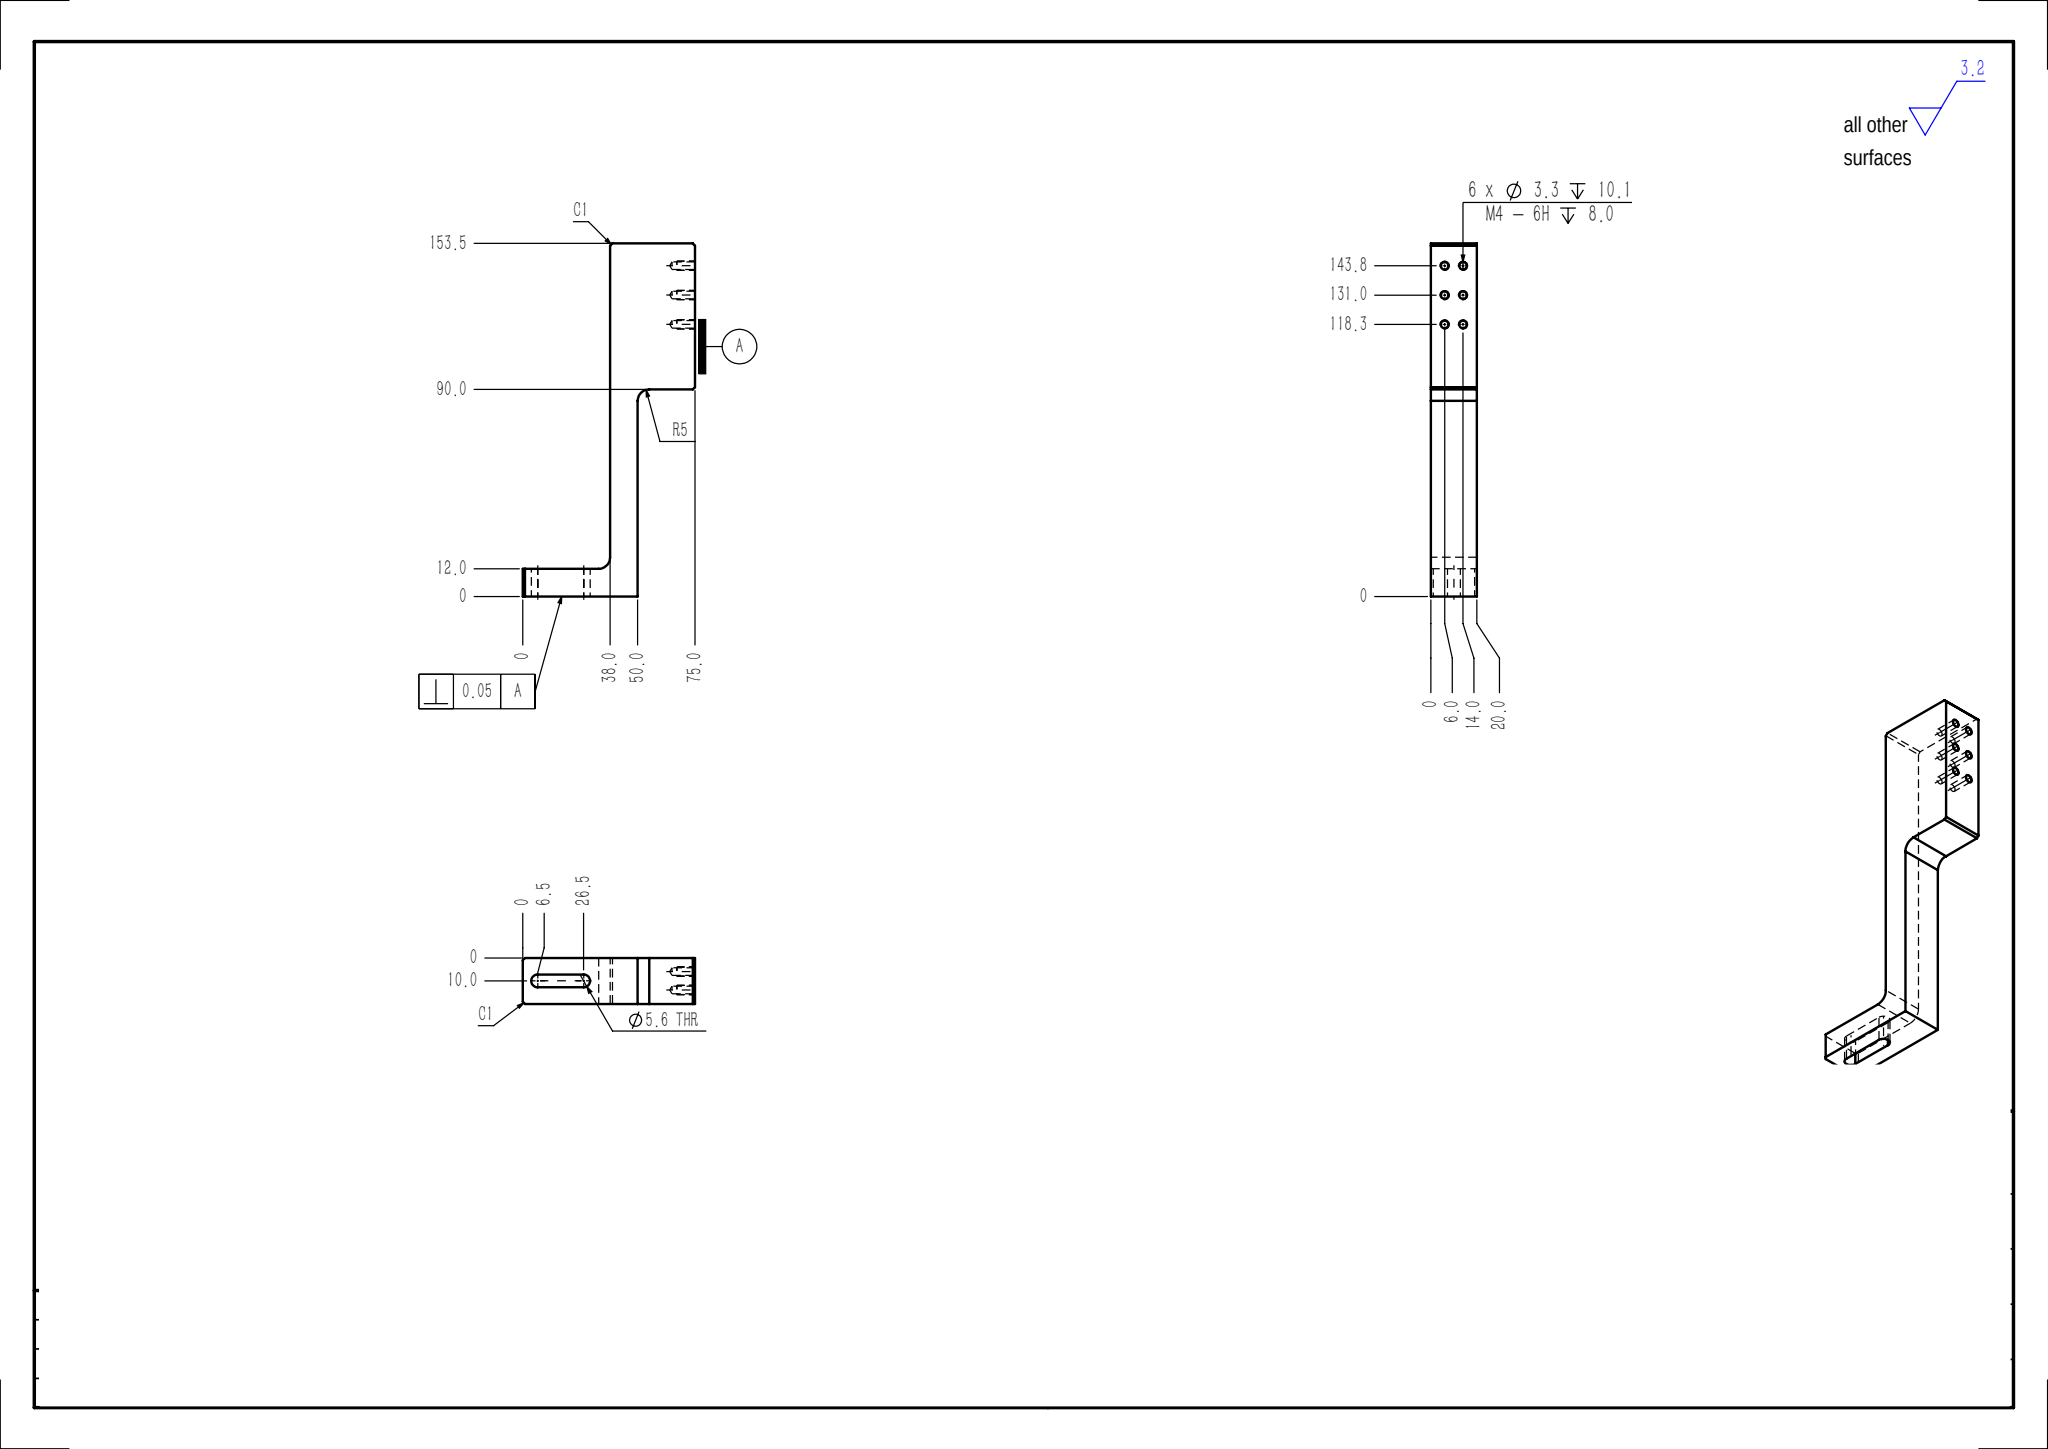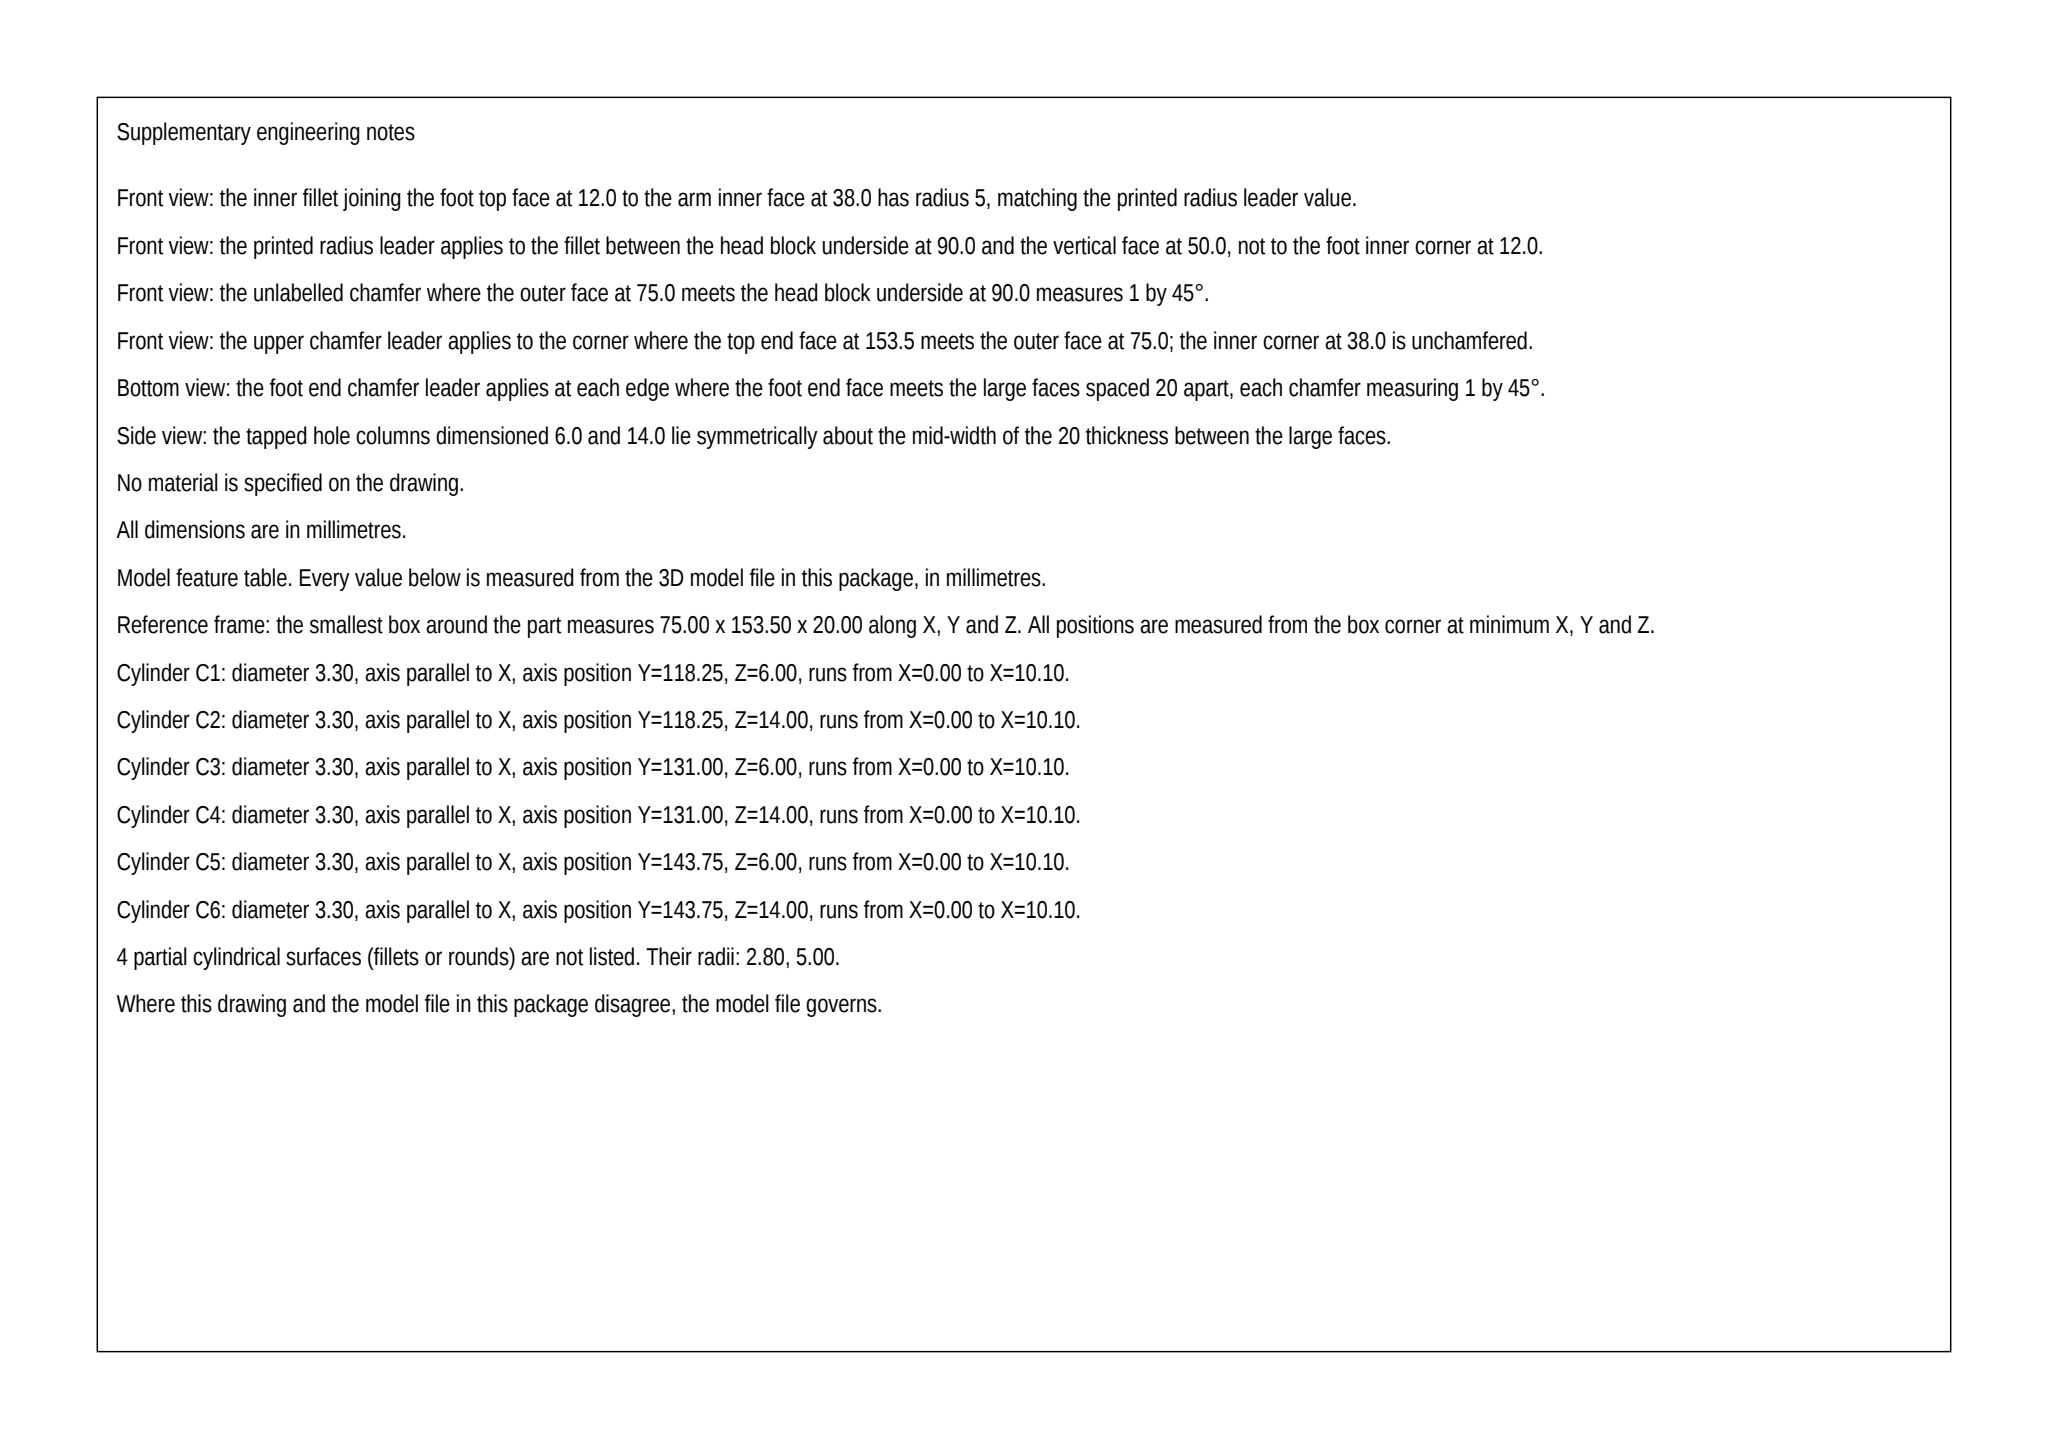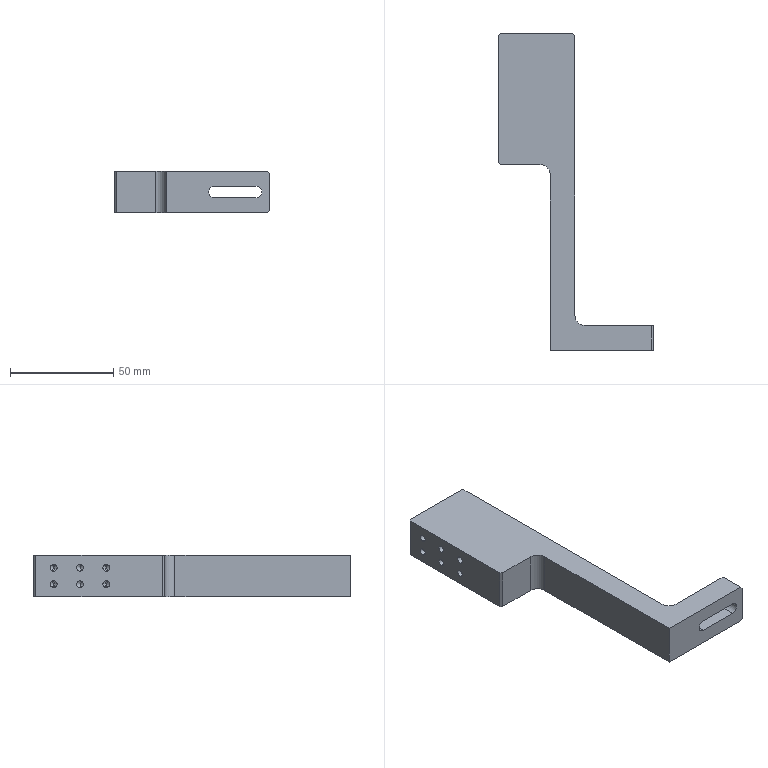Part | SolidWorks | mm | 1 solid | 45 faces | box 75 x 153.5 x 20 mm | volume 75708 mm3 | plane 17 | cylinder 16 | cone 12 | commonest cylinder face diameters 3.3 x12 10 x2 5.6 x2
Drawing notes:
2 X Ø5.6 THRU | from the solid: cylinders dia 5.6, axis y, len 12.0 = full y thickness (y planes 0 & 12.0), at x=48.5 & 68.5, z=10.0
build123d program:
from build123d import *

# Parameters (mm, degrees)
BOSS_EXTRUDE1_DEPTH   = 10
FILLET1_R             = 5
FILLET2_R             = 5
CUT_EXTRUDE1_DEPTH    = 151.407
CHAMFER1_SIZE         = 1
M4_TAPPED_HOLE1_D     = 3.3
M4_TAPPED_HOLE1_DEPTH = 10.1
M4_TAPPED_HOLE1_TIP   = 0.9914


with BuildPart() as part:
    # Sketch1 → Boss-Extrude1 (new, symmetric)
    with BuildSketch(Plane.XY):
        Polygon((-13, 76.75), (-13, -64.75), (25, -64.75), (25, -76.75), (-25, -76.75), (-25, 13.25), (-50, 13.25), (-50, 76.75), align=None)
    extrude(amount=BOSS_EXTRUDE1_DEPTH, both=True)

    # Fillet1
    fillet1_edges = [part.edges().sort_by_distance(p)[0] for p in [
        (-13, -64.75, 0),
    ]]
    fillet(fillet1_edges, radius=FILLET1_R)

    # Fillet2
    fillet2_edges = [part.edges().sort_by_distance(p)[0] for p in [
        (-25, 13.25, 0),
    ]]
    fillet(fillet2_edges, radius=FILLET2_R)

    # Sketch2 → Cut-Extrude1 (cut, through all)
    with BuildSketch(Plane(origin=(0, -64.75, 0), x_dir=(1, 0, 0), z_dir=(0, 1, 0))):
        with BuildLine():
            Line((-1.5, 2.8), (18.5, 2.8))
            ThreePointArc((18.5, 2.8), (21.3, 0), (18.5, -2.8))
            Line((18.5, -2.8), (-1.5, -2.8))
            ThreePointArc((-1.5, -2.8), (-4.3, 0), (-1.5, 2.8))
        make_face()
    extrude(amount=-CUT_EXTRUDE1_DEPTH, mode=Mode.SUBTRACT)

    # Chamfer1
    chamfer1_edges = [part.edges().sort_by_distance(p)[0] for p in [
        (25, -70.75, 10),
        (-50, 13.25, 0),
        (-50, 76.75, 0),
        (-13, 76.75, 0),
        (25, -70.75, -10),
    ]]
    chamfer(chamfer1_edges, length=CHAMFER1_SIZE)

    # M4 Tapped Hole1
    with Locations(Plane.ZY.offset(50)):
        with Locations((4, 67), (4, 41.5), (4, 54.25), (-4, 54.25), (-4, 41.5), (-4, 67)):
            Hole(M4_TAPPED_HOLE1_D / 2, depth=M4_TAPPED_HOLE1_DEPTH)
            with Locations((0, 0, -(M4_TAPPED_HOLE1_DEPTH + M4_TAPPED_HOLE1_TIP / 2))):  # 118° drill point
                Cone(0, M4_TAPPED_HOLE1_D / 2, M4_TAPPED_HOLE1_TIP, mode=Mode.SUBTRACT)


solid = part.part